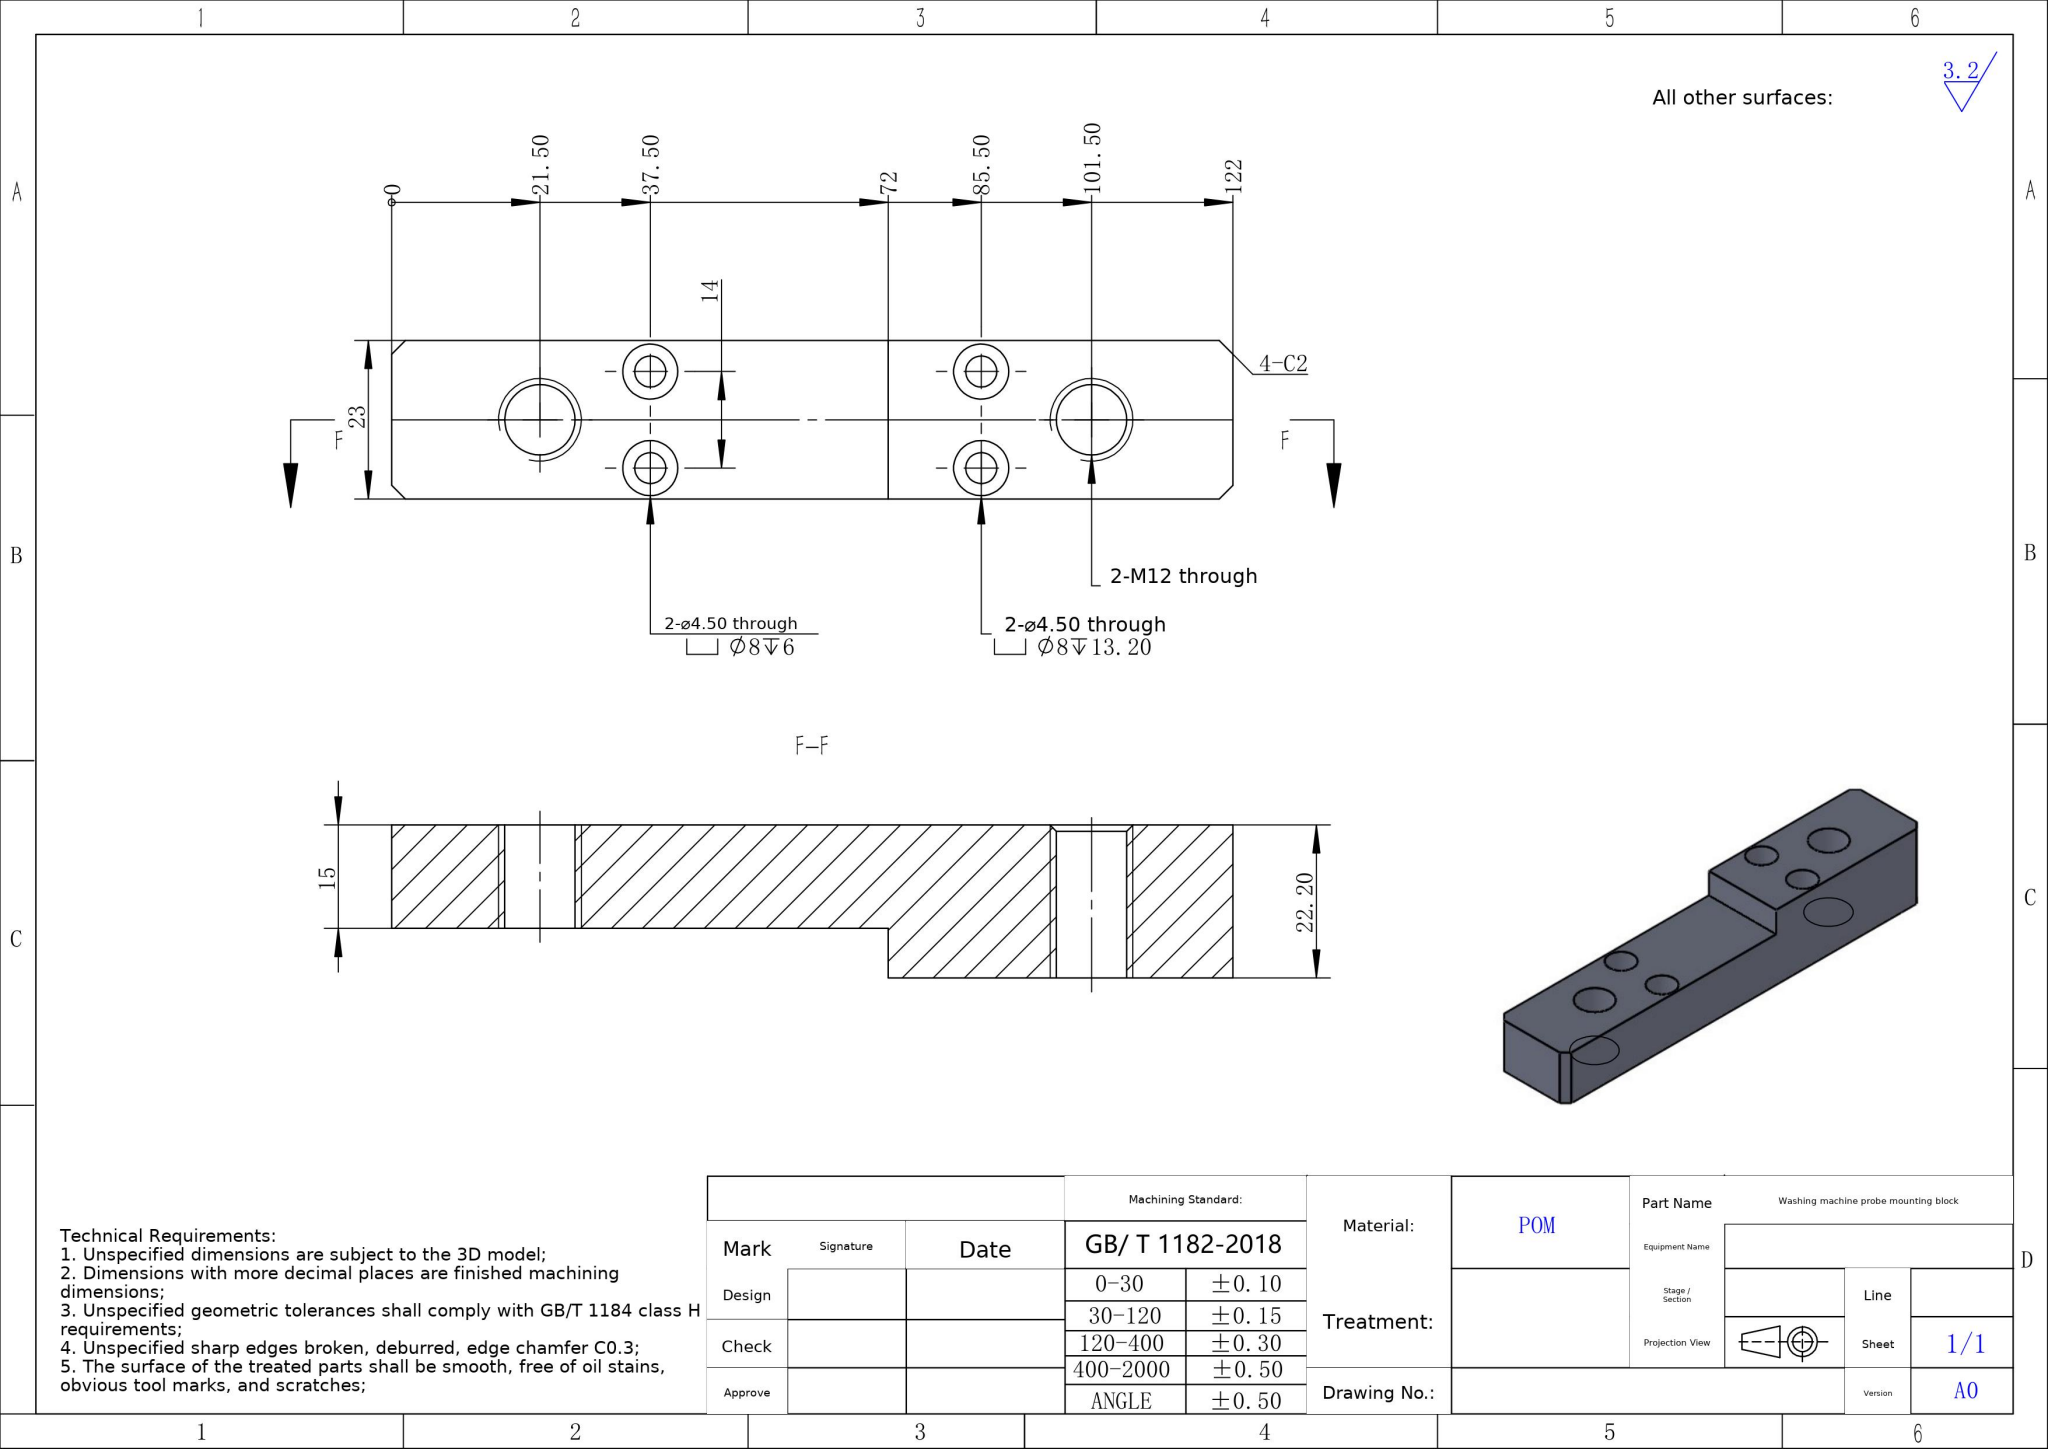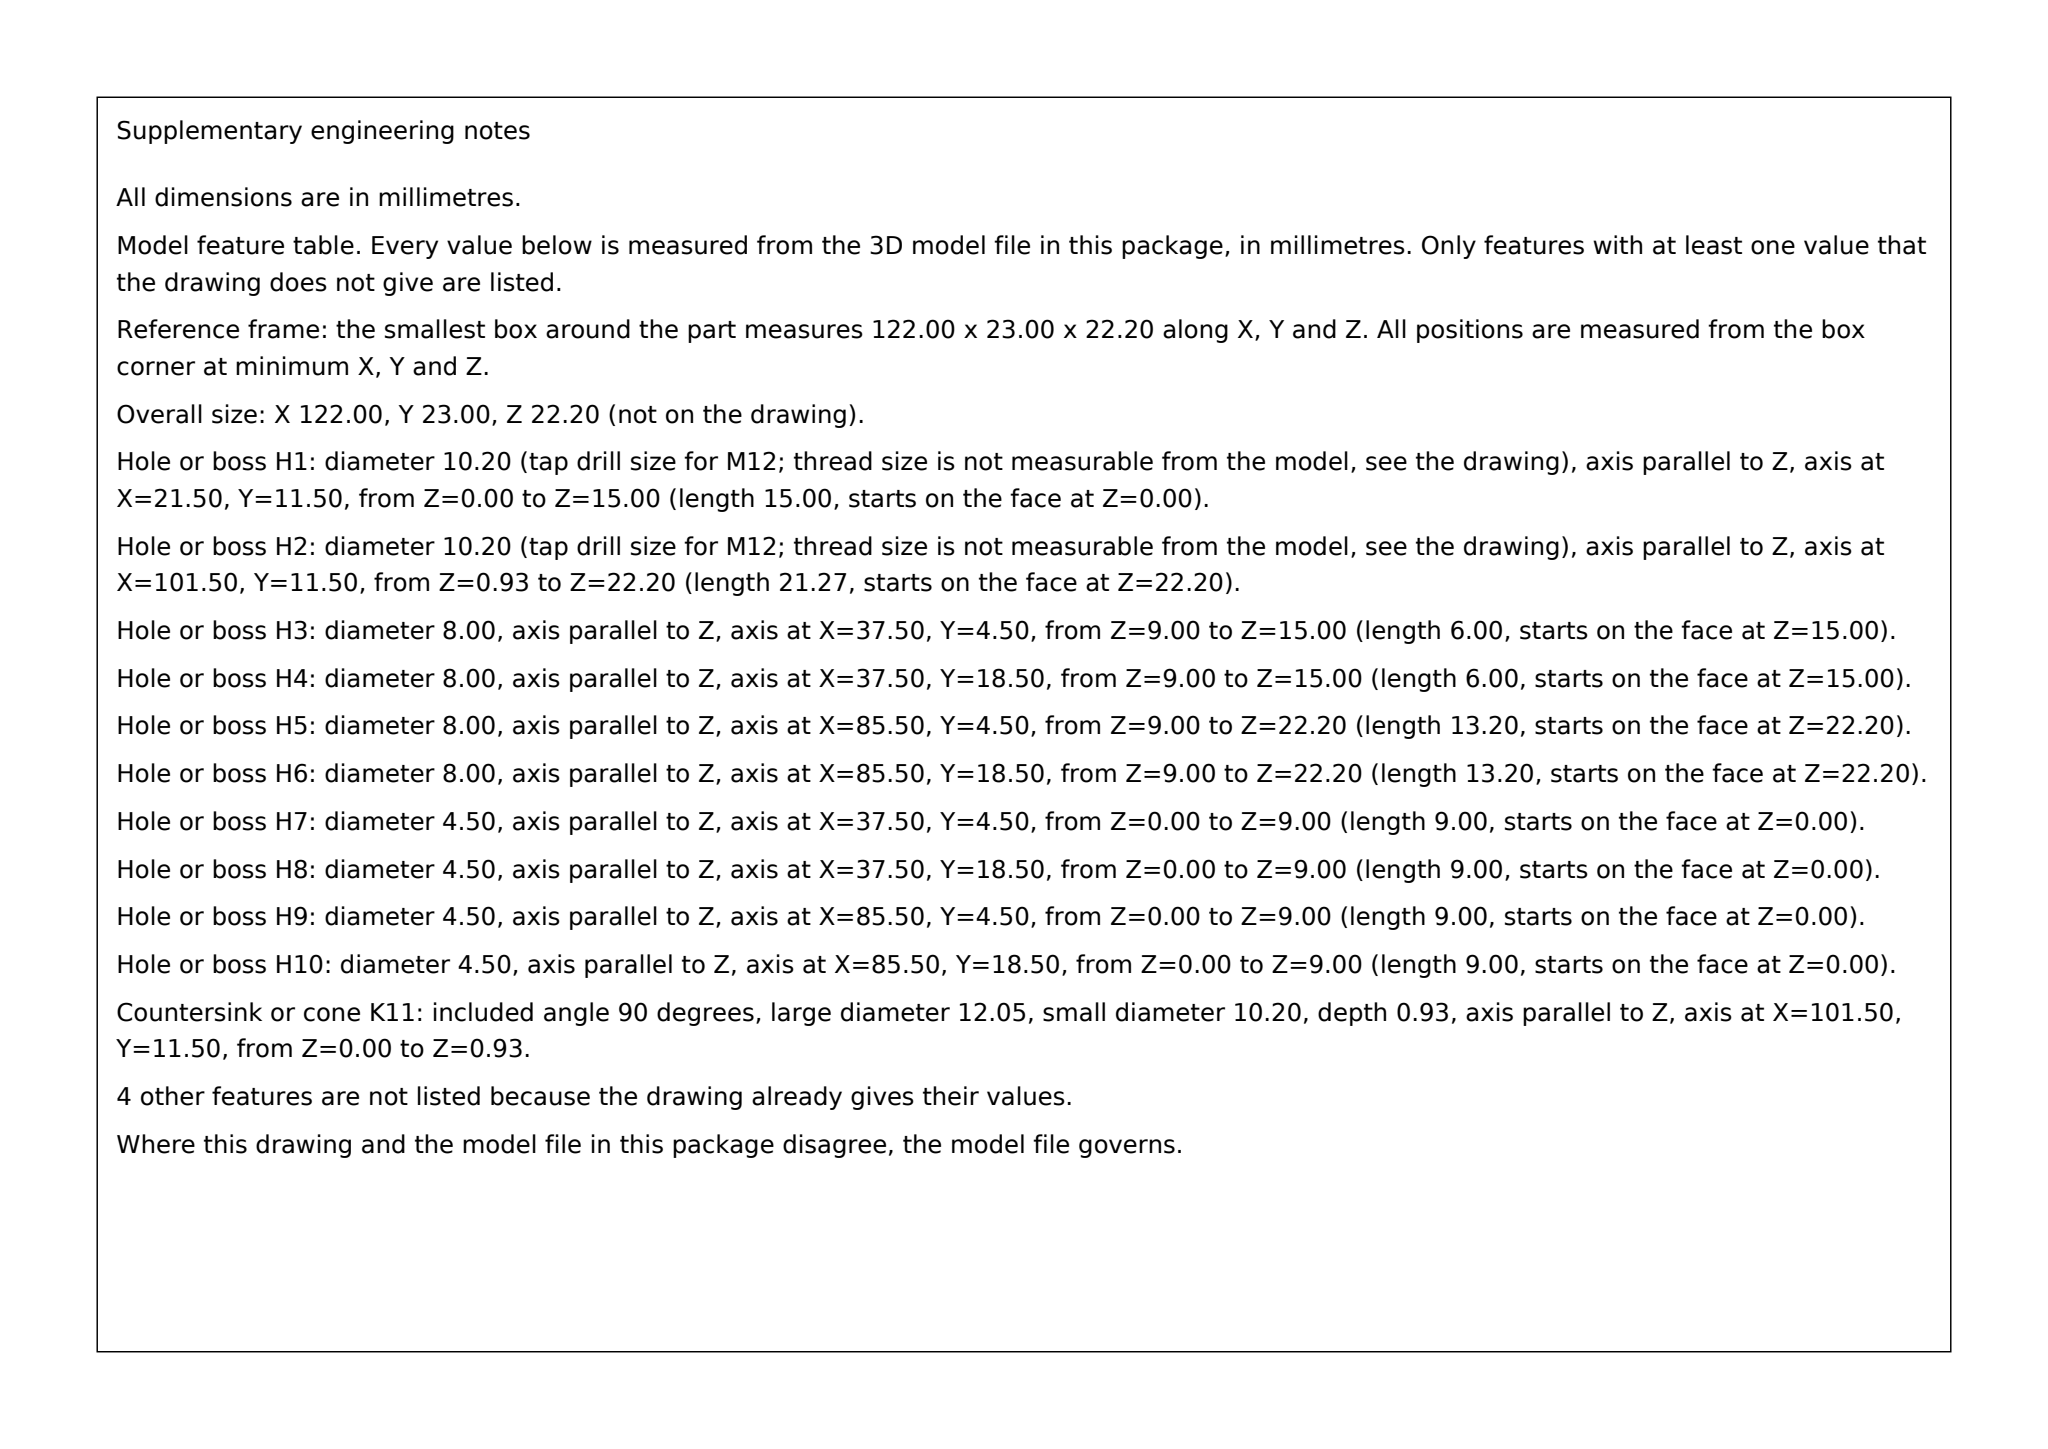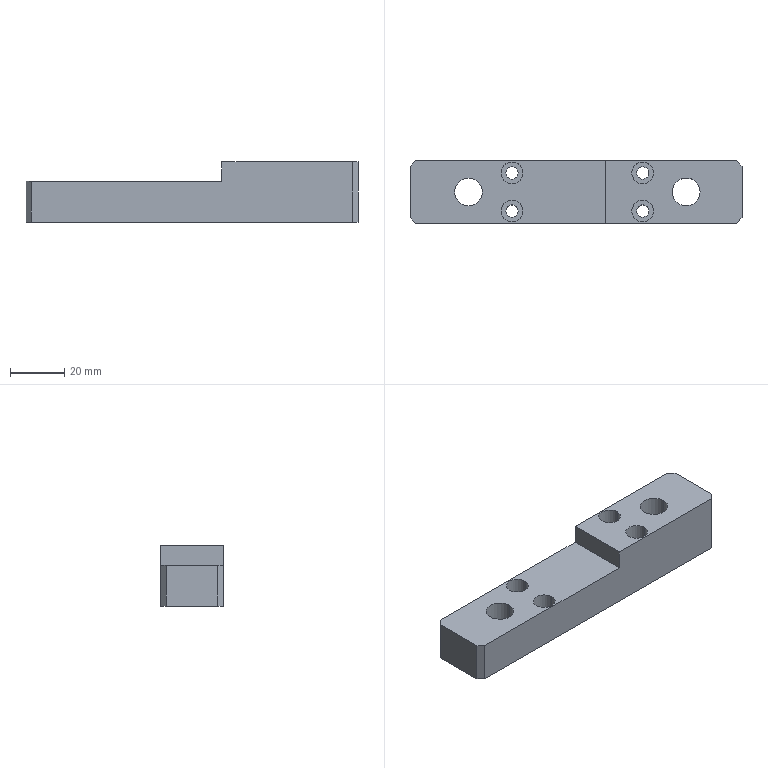Part | SolidWorks | mm | material POM | 1 solid | 38 faces | box 122 x 23 x 22.2 mm | volume 44664 mm3 | cylinder 20 | plane 16 | cone 2 | commonest cylinder face diameters 8 x8 4.5 x8 10.2 x4